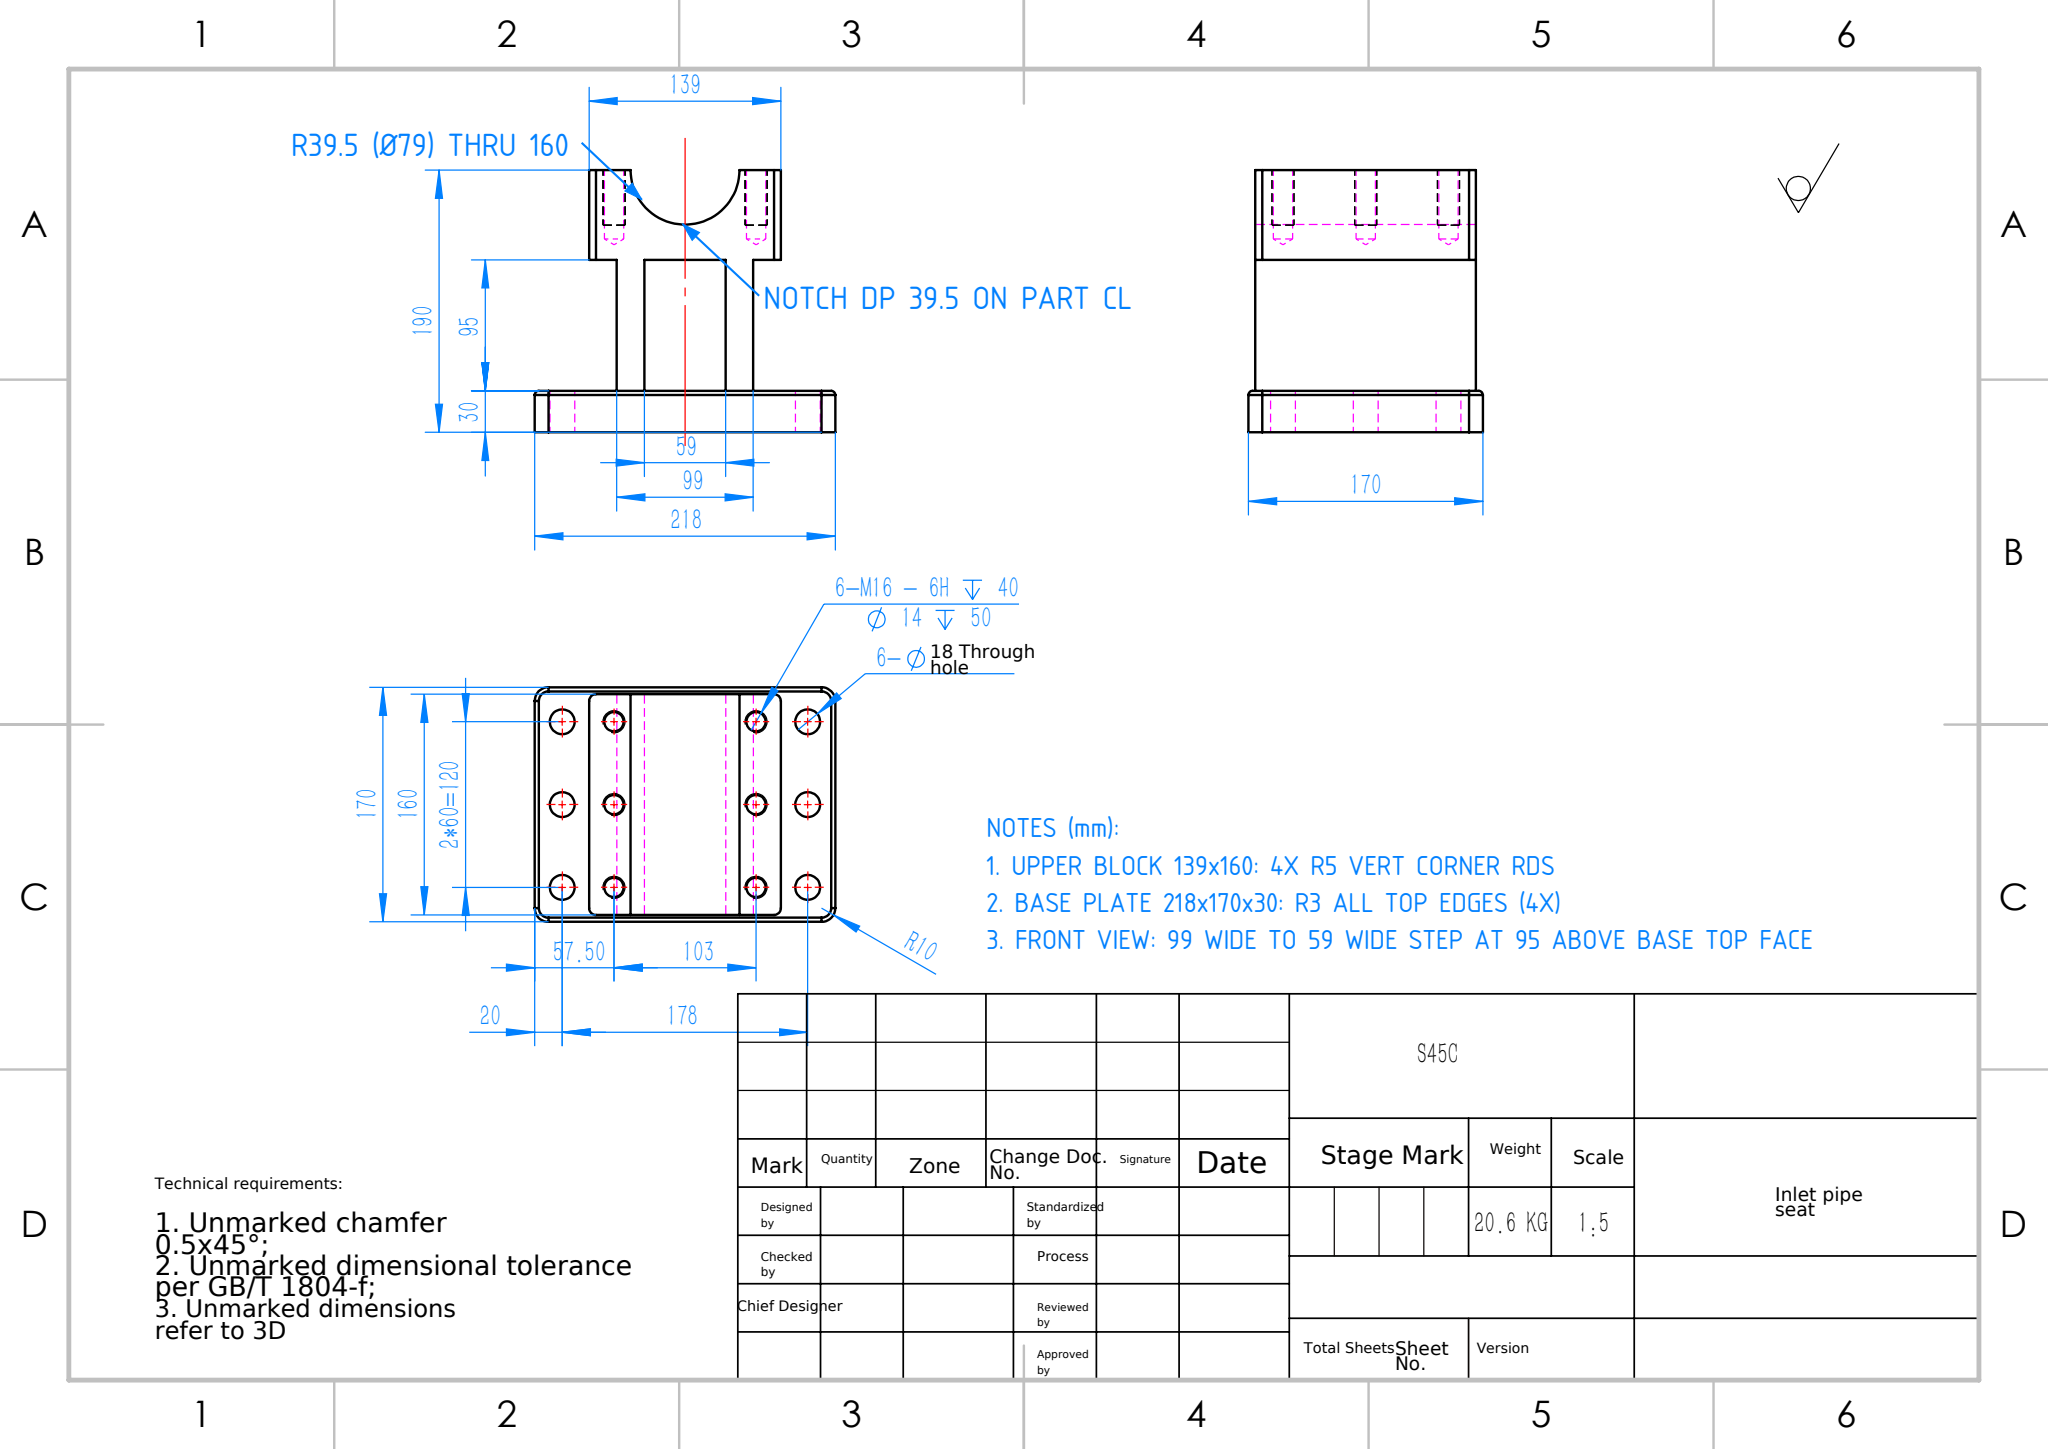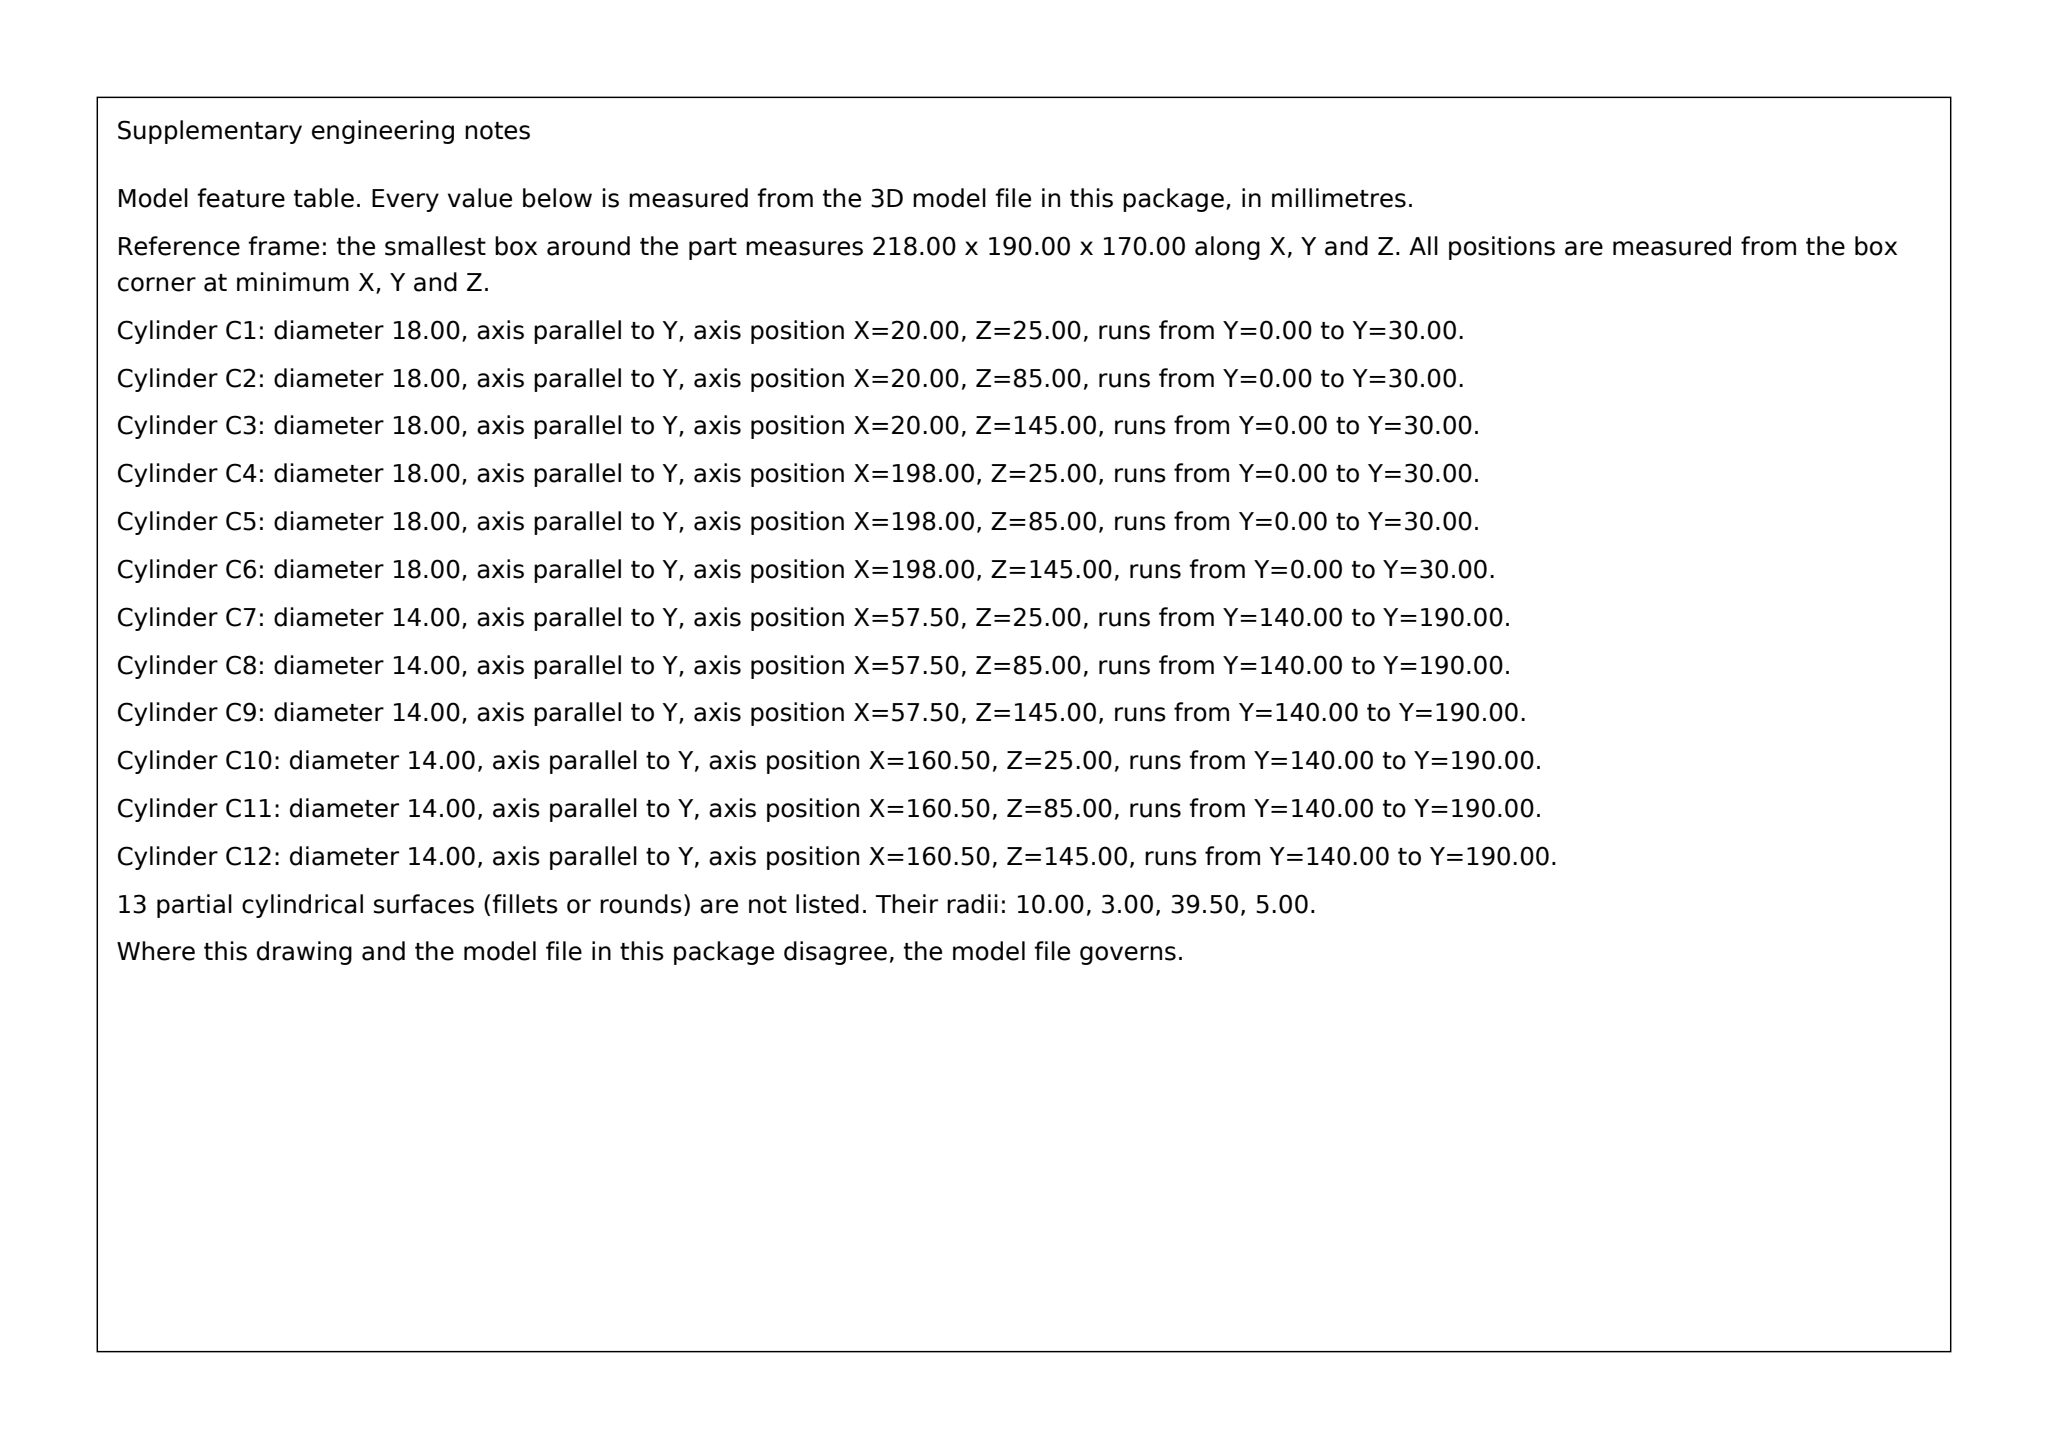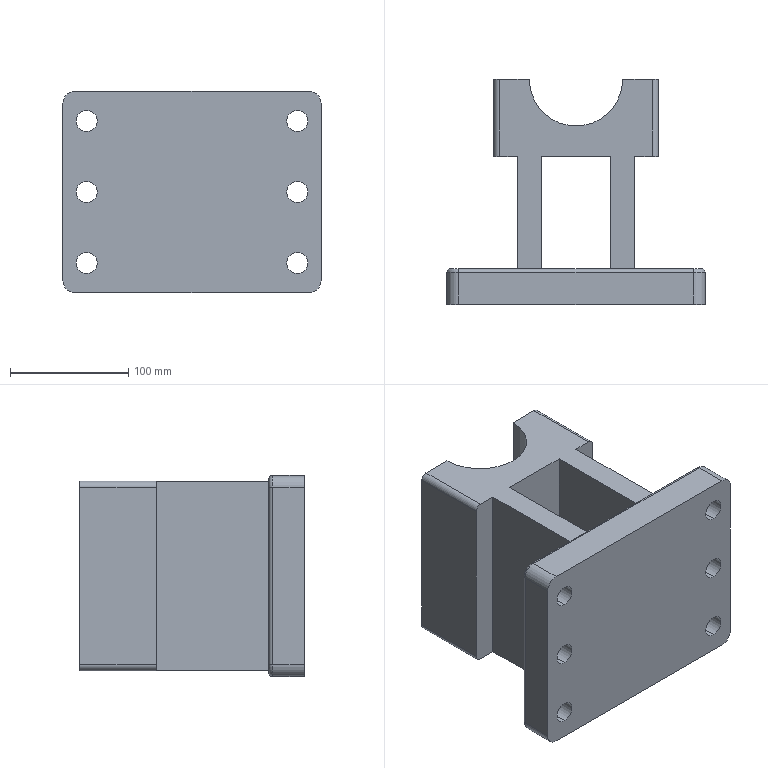Part | SolidWorks | mm | material S45C | 1 solid | 72 faces | box 218 x 190 x 170 mm | volume 2674558 mm3 | cylinder 37 | plane 19 | cone 12 | torus 4 | commonest cylinder face diameters 14 x12 18 x12 20 x4 6 x4 10 x4 79 x1
Drawing notes:
FRONT VIEW: TOP U-NOTCH R39.5 (Ø79) THRU 160 WIDTH | from the solid: cylinder dia 79.0, axis z, pos x=109.82 y=190.0, length 160
U-NOTCH AXIS ON 190 TOP FACE & ON PART CL, DEPTH 39.5 | from the solid: dia 79 cyl axis at y=190.0 (top face), x=109.82 = CL of 218/170 body
UPPER BLOCK 139x160: 4X R5 VERT CORNER RDS | from the solid: 4 cylinders dia 10.0, axis y, at x=45.32/174.32, z=10.82/160.82, len 65
BASE PLATE 218x170x30: R3 ALL TOP EDGES (4X) | from the solid: fillet_radii [3.0, 4]
FRONT VIEW: 99 WIDE TO 59 WIDE STEP AT 95 ABOVE BASE TOP FACE | from the solid: y-planes at 30 (base top) and 125 (only intermediate horiz face); x-planes 60.32/159.32 = 99 wide, 80.32/139.32 = 59 wide; 125-30 = 95
build123d program:
from build123d import *

# Parameters (mm, degrees)
SKETCH1_W                  = 218
SKETCH1_H                  = 170
EXTRUDE1_DEPTH             = 30
SKETCH2_W                  = 20
SKETCH2_H                  = 160
EXTRUDE2_DEPTH             = 95
EXTRUDE4_DEPTH             = 80
FILLET4_R                  = 10
FILLET5_R                  = 3
F_18_0_18_DIAMETER_HOLE1_D = 18
M16_TAPPED_HOLE1_D         = 14
M16_TAPPED_HOLE1_DEPTH     = 50
M16_TAPPED_HOLE1_TIP       = 4.206
FILLET6_R                  = 5


with BuildPart() as part:
    # Sketch1 → Extrude1 (new body)
    with BuildSketch(Plane(origin=(0, 0, 0), x_dir=(1, 0, 0), z_dir=(0, 1, 0))):
        Rectangle(SKETCH1_W, SKETCH1_H)
    extrude(amount=EXTRUDE1_DEPTH)

    # Sketch2 → Extrude2 (add)
    with BuildSketch(Plane(origin=(0, 30, 0), x_dir=(1, 0, 0), z_dir=(0, 1, 0))):
        with Locations((-39.5, 0)):
            Rectangle(SKETCH2_W, SKETCH2_H)
        with Locations((39.5, 0)):
            Rectangle(SKETCH2_W, SKETCH2_H)
    extrude(amount=EXTRUDE2_DEPTH)

    # Sketch4 → Extrude4 (add, symmetric)
    with BuildSketch(Plane.XY):
        with BuildLine():
            Line((-69.5, 190), (-39.5, 190))
            ThreePointArc((-39.5, 190), (0, 150.5), (39.5, 190))
            Line((39.5, 190), (69.5, 190))
            Line((69.5, 190), (69.5, 125))
            Line((69.5, 125), (-69.5, 125))
            Line((-69.5, 125), (-69.5, 190))
        make_face()
    extrude(amount=EXTRUDE4_DEPTH, both=True)

    # Fillet4
    fillet4_edges = [part.edges().sort_by_distance(p)[0] for p in [
        (109, 15, 85),
        (-109, 15, 85),
        (-109, 15, -85),
        (109, 15, -85),
    ]]
    fillet(fillet4_edges, radius=FILLET4_R)

    # Fillet5
    fillet5_edges = [part.edges().sort_by_distance(p)[0] for p in [
        (-109, 30, 0),
        (0, 30, -85),
        (109, 30, 0),
        (0, 30, 85),
        (-106.071, 30, 82.071),
        (106.071, 30, 82.071),
        (106.071, 30, -82.071),
        (-106.071, 30, -82.071),
    ]]
    fillet(fillet5_edges, radius=FILLET5_R)

    # 18.0 _18_ Diameter Hole1 (through all)
    with Locations(Plane(origin=(0, 30, 0), x_dir=(-1, 0, 0), z_dir=(0, 1, 0))):
        with Locations((89, 60), (89, -60), (-89, -60), (-89, 60), (-89, 0), (89, 0)):
            Hole(F_18_0_18_DIAMETER_HOLE1_D / 2)

    # M16 Tapped Hole1
    with Locations(Plane(origin=(0, 190, 0), x_dir=(-1, 0, 0), z_dir=(0, 1, 0))):
        with Locations((51.5, -60), (51.5, 60), (-51.5, -60), (-51.5, 60), (-51.5, 0), (51.5, 0)):
            Hole(M16_TAPPED_HOLE1_D / 2, depth=M16_TAPPED_HOLE1_DEPTH)
            with Locations((0, 0, -(M16_TAPPED_HOLE1_DEPTH + M16_TAPPED_HOLE1_TIP / 2))):  # 118° drill point
                Cone(0, M16_TAPPED_HOLE1_D / 2, M16_TAPPED_HOLE1_TIP, mode=Mode.SUBTRACT)

    # Fillet6
    fillet6_edges = [part.edges().sort_by_distance(p)[0] for p in [
        (69.5, 157.5, -80),
        (69.5, 157.5, 80),
        (-69.5, 157.5, -80),
        (-69.5, 157.5, 80),
    ]]
    fillet(fillet6_edges, radius=FILLET6_R)


solid = part.part